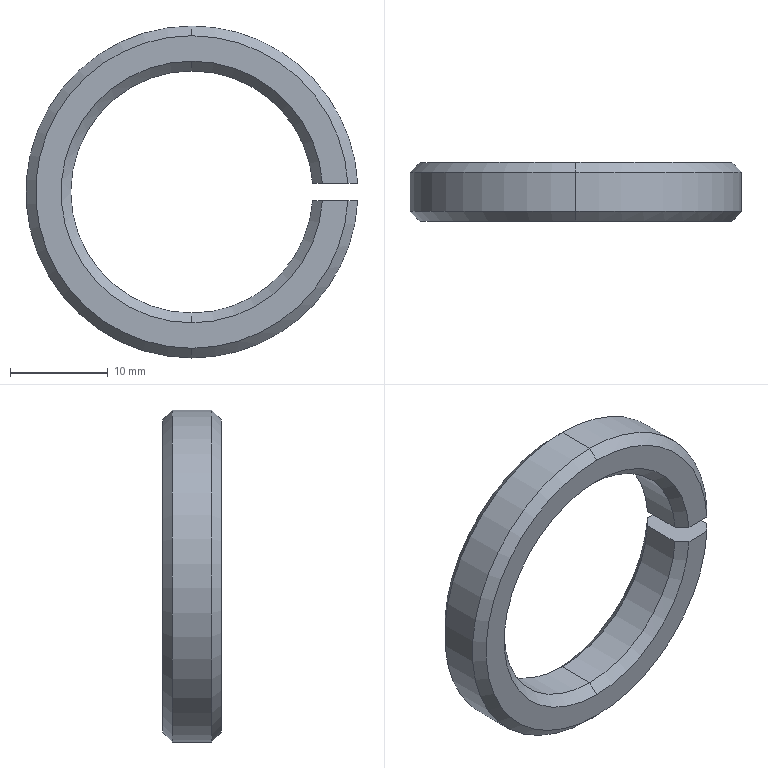Part | SolidWorks | mm | material Rubber | 1 solid | 22 faces | box 33.98 x 6 x 34 mm | volume 2318 mm3 | cone 12 | cylinder 6 | plane 4 | commonest cylinder face diameters 24.8 x3 34 x3
build123d program:
from build123d import *

# Parameters (mm, degrees)
SKETCH1_W          = 4.6
SKETCH1_H          = 6
CHAMFER1_SIZE      = 1
SKETCH2_W          = 15
SKETCH2_H          = 1.8
CUT_EXTRUDE1_DEPTH = 25.779


with BuildPart() as part:
    # Sketch1 → Revolve1 (revolve)
    with BuildSketch(Plane.XY, mode=Mode.PRIVATE) as revolve1_sk:
        with Locations((14.7, 0)):
            Rectangle(SKETCH1_W, SKETCH1_H)
    revolve(revolve1_sk.sketch.rotate(Axis((0, -27.466, 0), (0, 1, 0)), 90), axis=Axis((0, -27.466, 0), (0, 1, 0)))

    # Chamfer1
    chamfer1_edges = [part.edges().sort_by_distance(p)[0] for p in [
        (0, -3, 17),
        (0, -3, 12.4),
        (0, 3, 12.4),
        (0, 3, 17),
    ]]
    chamfer(chamfer1_edges, length=CHAMFER1_SIZE)

    # Sketch2 → Cut-Extrude1 (cut, through all)
    with BuildSketch(Plane(origin=(0, 3, 0), x_dir=(1, 0, 0), z_dir=(0, 1, 0))):
        with Locations((15.5, 0)):
            Rectangle(SKETCH2_W, SKETCH2_H)
    extrude(amount=-CUT_EXTRUDE1_DEPTH, mode=Mode.SUBTRACT)


solid = part.part
STEP:
#1=CARTESIAN_POINT('',(0.,3.,16.));
#2=VERTEX_POINT('',#1);
#3=CARTESIAN_POINT('',(15.975,3.,0.9));
#4=VERTEX_POINT('',#3);
#5=CARTESIAN_POINT('',(0.,3.,0.));
#6=DIRECTION('',(0.,1.,0.));
#7=DIRECTION('',(0.,0.,-1.));
#8=AXIS2_PLACEMENT_3D('',#5,#6,#7);
#9=CIRCLE('',#8,16.);
#10=EDGE_CURVE('',#2,#4,#9,.T.);
#11=ORIENTED_EDGE('',*,*,#10,.F.);
#12=CARTESIAN_POINT('',(0.,2.,17.));
#13=VERTEX_POINT('',#12);
#14=CARTESIAN_POINT('',(0.,2.,17.));
#15=DIRECTION('',(0.,-0.7071,0.7071));
#16=VECTOR('',#15,1000.);
#17=LINE('',#14,#16);
#18=EDGE_CURVE('',#2,#13,#17,.T.);
#19=ORIENTED_EDGE('',*,*,#18,.T.);
#20=CARTESIAN_POINT('',(16.976,2.,0.9));
#21=VERTEX_POINT('',#20);
#22=CARTESIAN_POINT('',(0.,2.,0.));
#23=DIRECTION('',(0.,-1.,0.));
#24=DIRECTION('',(0.,0.,-1.));
#25=AXIS2_PLACEMENT_3D('',#22,#23,#24);
#26=CIRCLE('',#25,17.);
#27=EDGE_CURVE('',#21,#13,#26,.T.);
#28=ORIENTED_EDGE('',*,*,#27,.F.);
#29=CARTESIAN_POINT('',(15.975,3.,0.9));
#30=CARTESIAN_POINT('',(16.309,2.667,0.9));
#31=CARTESIAN_POINT('',(16.642,2.333,0.9));
#32=CARTESIAN_POINT('',(16.976,2.,0.9));
#33=B_SPLINE_CURVE_WITH_KNOTS('',3,(#29,#30,#31,#32),.UNSPECIFIED.,.F.,.F.,(4,4),(0.01619,0.01761),.UNSPECIFIED.);
#34=EDGE_CURVE('',#4,#21,#33,.T.);
#35=ORIENTED_EDGE('',*,*,#34,.F.);
#36=EDGE_LOOP('',(#11,#19,#28,#35));
#37=FACE_OUTER_BOUND('',#36,.T.);
#38=CARTESIAN_POINT('',(0.,2.,0.));
#39=DIRECTION('',(0.,-1.,0.));
#40=DIRECTION('',(0.,0.,-1.));
#41=AXIS2_PLACEMENT_3D('',#38,#39,#40);
#42=CONICAL_SURFACE('',#41,17.,0.7854);
#43=ADVANCED_FACE('',(#37),#42,.T.);
#44=ORIENTED_EDGE('',*,*,#18,.F.);
#45=CARTESIAN_POINT('',(0.,3.,-16.));
#46=VERTEX_POINT('',#45);
#47=CARTESIAN_POINT('',(0.,3.,0.));
#48=DIRECTION('',(0.,1.,0.));
#49=DIRECTION('',(0.,0.,-1.));
#50=AXIS2_PLACEMENT_3D('',#47,#48,#49);
#51=CIRCLE('',#50,16.);
#52=EDGE_CURVE('',#46,#2,#51,.T.);
#53=ORIENTED_EDGE('',*,*,#52,.F.);
#54=CARTESIAN_POINT('',(0.,2.,-17.));
#55=VERTEX_POINT('',#54);
#56=CARTESIAN_POINT('',(0.,2.,-17.));
#57=DIRECTION('',(0.,-0.7071,-0.7071));
#58=VECTOR('',#57,1000.);
#59=LINE('',#56,#58);
#60=EDGE_CURVE('',#46,#55,#59,.T.);
#61=ORIENTED_EDGE('',*,*,#60,.T.);
#62=CARTESIAN_POINT('',(0.,2.,0.));
#63=DIRECTION('',(0.,-1.,0.));
#64=DIRECTION('',(0.,0.,-1.));
#65=AXIS2_PLACEMENT_3D('',#62,#63,#64);
#66=CIRCLE('',#65,17.);
#67=EDGE_CURVE('',#13,#55,#66,.T.);
#68=ORIENTED_EDGE('',*,*,#67,.F.);
#69=EDGE_LOOP('',(#44,#53,#61,#68));
#70=FACE_OUTER_BOUND('',#69,.T.);
#71=CARTESIAN_POINT('',(0.,2.,0.));
#72=DIRECTION('',(0.,-1.,0.));
#73=DIRECTION('',(0.,0.,-1.));
#74=AXIS2_PLACEMENT_3D('',#71,#72,#73);
#75=CONICAL_SURFACE('',#74,17.,0.7854);
#76=ADVANCED_FACE('',(#70),#75,.T.);
#77=CARTESIAN_POINT('',(0.,-3.,-16.));
#78=VERTEX_POINT('',#77);
#79=CARTESIAN_POINT('',(15.975,-3.,-0.9));
#80=VERTEX_POINT('',#79);
#81=CARTESIAN_POINT('',(0.,-3.,0.));
#82=DIRECTION('',(0.,-1.,0.));
#83=DIRECTION('',(0.,0.,-1.));
#84=AXIS2_PLACEMENT_3D('',#81,#82,#83);
#85=CIRCLE('',#84,16.);
#86=EDGE_CURVE('',#78,#80,#85,.T.);
#87=ORIENTED_EDGE('',*,*,#86,.F.);
#88=CARTESIAN_POINT('',(0.,-2.,-17.));
#89=VERTEX_POINT('',#88);
#90=CARTESIAN_POINT('',(0.,-3.,-16.));
#91=DIRECTION('',(0.,0.7071,-0.7071));
#92=VECTOR('',#91,1000.);
#93=LINE('',#90,#92);
#94=EDGE_CURVE('',#78,#89,#93,.T.);
#95=ORIENTED_EDGE('',*,*,#94,.T.);
#96=CARTESIAN_POINT('',(16.976,-2.,-0.9));
#97=VERTEX_POINT('',#96);
#98=CARTESIAN_POINT('',(0.,-2.,0.));
#99=DIRECTION('',(0.,1.,0.));
#100=DIRECTION('',(-0.,0.,-1.));
#101=AXIS2_PLACEMENT_3D('',#98,#99,#100);
#102=CIRCLE('',#101,17.);
#103=EDGE_CURVE('',#97,#89,#102,.T.);
#104=ORIENTED_EDGE('',*,*,#103,.F.);
#105=CARTESIAN_POINT('',(15.975,-3.,-0.9));
#106=CARTESIAN_POINT('',(16.309,-2.667,-0.9));
#107=CARTESIAN_POINT('',(16.642,-2.333,-0.9));
#108=CARTESIAN_POINT('',(16.976,-2.,-0.9));
#109=B_SPLINE_CURVE_WITH_KNOTS('',3,(#105,#106,#107,#108),.UNSPECIFIED.,.F.,.F.,(4,4),(0.01619,0.01761),.UNSPECIFIED.);
#110=EDGE_CURVE('',#80,#97,#109,.T.);
#111=ORIENTED_EDGE('',*,*,#110,.F.);
#112=EDGE_LOOP('',(#87,#95,#104,#111));
#113=FACE_OUTER_BOUND('',#112,.T.);
#114=CARTESIAN_POINT('',(0.,-3.,0.));
#115=DIRECTION('',(0.,1.,0.));
#116=DIRECTION('',(0.,0.,1.));
#117=AXIS2_PLACEMENT_3D('',#114,#115,#116);
#118=CONICAL_SURFACE('',#117,16.,0.7854);
#119=ADVANCED_FACE('',(#113),#118,.T.);
#120=ORIENTED_EDGE('',*,*,#94,.F.);
#121=CARTESIAN_POINT('',(0.,-3.,16.));
#122=VERTEX_POINT('',#121);
#123=CARTESIAN_POINT('',(0.,-3.,0.));
#124=DIRECTION('',(0.,-1.,0.));
#125=DIRECTION('',(0.,0.,-1.));
#126=AXIS2_PLACEMENT_3D('',#123,#124,#125);
#127=CIRCLE('',#126,16.);
#128=EDGE_CURVE('',#122,#78,#127,.T.);
#129=ORIENTED_EDGE('',*,*,#128,.F.);
#130=CARTESIAN_POINT('',(0.,-2.,17.));
#131=VERTEX_POINT('',#130);
#132=CARTESIAN_POINT('',(0.,-3.,16.));
#133=DIRECTION('',(0.,0.7071,0.7071));
#134=VECTOR('',#133,1000.);
#135=LINE('',#132,#134);
#136=EDGE_CURVE('',#122,#131,#135,.T.);
#137=ORIENTED_EDGE('',*,*,#136,.T.);
#138=CARTESIAN_POINT('',(0.,-2.,0.));
#139=DIRECTION('',(0.,1.,0.));
#140=DIRECTION('',(0.,0.,-1.));
#141=AXIS2_PLACEMENT_3D('',#138,#139,#140);
#142=CIRCLE('',#141,17.);
#143=EDGE_CURVE('',#89,#131,#142,.T.);
#144=ORIENTED_EDGE('',*,*,#143,.F.);
#145=EDGE_LOOP('',(#120,#129,#137,#144));
#146=FACE_OUTER_BOUND('',#145,.T.);
#147=CARTESIAN_POINT('',(0.,-3.,0.));
#148=DIRECTION('',(0.,1.,0.));
#149=DIRECTION('',(0.,0.,1.));
#150=AXIS2_PLACEMENT_3D('',#147,#148,#149);
#151=CONICAL_SURFACE('',#150,16.,0.7854);
#152=ADVANCED_FACE('',(#146),#151,.T.);
#153=CARTESIAN_POINT('',(0.,2.,-12.4));
#154=VERTEX_POINT('',#153);
#155=CARTESIAN_POINT('',(0.,2.,12.4));
#156=VERTEX_POINT('',#155);
#157=CARTESIAN_POINT('',(0.,2.,0.));
#158=DIRECTION('',(0.,1.,0.));
#159=DIRECTION('',(0.,0.,-1.));
#160=AXIS2_PLACEMENT_3D('',#157,#158,#159);
#161=CIRCLE('',#160,12.4);
#162=EDGE_CURVE('',#154,#156,#161,.T.);
#163=ORIENTED_EDGE('',*,*,#162,.F.);
#164=CARTESIAN_POINT('',(0.,3.,-13.4));
#165=VERTEX_POINT('',#164);
#166=CARTESIAN_POINT('',(0.,3.,-13.4));
#167=DIRECTION('',(0.,0.7071,-0.7071));
#168=VECTOR('',#167,1000.);
#169=LINE('',#166,#168);
#170=EDGE_CURVE('',#154,#165,#169,.T.);
#171=ORIENTED_EDGE('',*,*,#170,.T.);
#172=CARTESIAN_POINT('',(0.,3.,13.4));
#173=VERTEX_POINT('',#172);
#174=CARTESIAN_POINT('',(0.,3.,0.));
#175=DIRECTION('',(0.,-1.,0.));
#176=DIRECTION('',(0.,0.,-1.));
#177=AXIS2_PLACEMENT_3D('',#174,#175,#176);
#178=CIRCLE('',#177,13.4);
#179=EDGE_CURVE('',#173,#165,#178,.T.);
#180=ORIENTED_EDGE('',*,*,#179,.F.);
#181=CARTESIAN_POINT('',(0.,3.,13.4));
#182=DIRECTION('',(0.,0.7071,0.7071));
#183=VECTOR('',#182,1000.);
#184=LINE('',#181,#183);
#185=EDGE_CURVE('',#156,#173,#184,.T.);
#186=ORIENTED_EDGE('',*,*,#185,.F.);
#187=EDGE_LOOP('',(#163,#171,#180,#186));
#188=FACE_OUTER_BOUND('',#187,.T.);
#189=CARTESIAN_POINT('',(0.,3.,0.));
#190=DIRECTION('',(0.,1.,0.));
#191=DIRECTION('',(0.,0.,1.));
#192=AXIS2_PLACEMENT_3D('',#189,#190,#191);
#193=CONICAL_SURFACE('',#192,13.4,0.7854);
#194=ADVANCED_FACE('',(#188),#193,.F.);
#195=CARTESIAN_POINT('',(12.367,2.,0.9));
#196=VERTEX_POINT('',#195);
#197=CARTESIAN_POINT('',(0.,2.,0.));
#198=DIRECTION('',(0.,1.,0.));
#199=DIRECTION('',(0.,0.,-1.));
#200=AXIS2_PLACEMENT_3D('',#197,#198,#199);
#201=CIRCLE('',#200,12.4);
#202=EDGE_CURVE('',#156,#196,#201,.T.);
#203=ORIENTED_EDGE('',*,*,#202,.F.);
#204=ORIENTED_EDGE('',*,*,#185,.T.);
#205=CARTESIAN_POINT('',(13.37,3.,0.9));
#206=VERTEX_POINT('',#205);
#207=CARTESIAN_POINT('',(0.,3.,0.));
#208=DIRECTION('',(0.,-1.,0.));
#209=DIRECTION('',(0.,0.,-1.));
#210=AXIS2_PLACEMENT_3D('',#207,#208,#209);
#211=CIRCLE('',#210,13.4);
#212=EDGE_CURVE('',#206,#173,#211,.T.);
#213=ORIENTED_EDGE('',*,*,#212,.F.);
#214=CARTESIAN_POINT('',(12.367,2.,0.9));
#215=CARTESIAN_POINT('',(12.701,2.333,0.9));
#216=CARTESIAN_POINT('',(13.036,2.667,0.9));
#217=CARTESIAN_POINT('',(13.37,3.,0.9));
#218=B_SPLINE_CURVE_WITH_KNOTS('',3,(#214,#215,#216,#217),.UNSPECIFIED.,.F.,.F.,(4,4),(0.009566,0.01098),.UNSPECIFIED.);
#219=EDGE_CURVE('',#196,#206,#218,.T.);
#220=ORIENTED_EDGE('',*,*,#219,.F.);
#221=EDGE_LOOP('',(#203,#204,#213,#220));
#222=FACE_OUTER_BOUND('',#221,.T.);
#223=CARTESIAN_POINT('',(0.,3.,0.));
#224=DIRECTION('',(0.,1.,0.));
#225=DIRECTION('',(0.,0.,1.));
#226=AXIS2_PLACEMENT_3D('',#223,#224,#225);
#227=CONICAL_SURFACE('',#226,13.4,0.7854);
#228=ADVANCED_FACE('',(#222),#227,.F.);
#229=CARTESIAN_POINT('',(0.,-2.,12.4));
#230=VERTEX_POINT('',#229);
#231=CARTESIAN_POINT('',(0.,-2.,-12.4));
#232=VERTEX_POINT('',#231);
#233=CARTESIAN_POINT('',(0.,-2.,0.));
#234=DIRECTION('',(0.,-1.,0.));
#235=DIRECTION('',(0.,0.,-1.));
#236=AXIS2_PLACEMENT_3D('',#233,#234,#235);
#237=CIRCLE('',#236,12.4);
#238=EDGE_CURVE('',#230,#232,#237,.T.);
#239=ORIENTED_EDGE('',*,*,#238,.F.);
#240=CARTESIAN_POINT('',(0.,-3.,13.4));
#241=VERTEX_POINT('',#240);
#242=CARTESIAN_POINT('',(0.,-2.,12.4));
#243=DIRECTION('',(0.,-0.7071,0.7071));
#244=VECTOR('',#243,1000.);
#245=LINE('',#242,#244);
#246=EDGE_CURVE('',#230,#241,#245,.T.);
#247=ORIENTED_EDGE('',*,*,#246,.T.);
#248=CARTESIAN_POINT('',(0.,-3.,-13.4));
#249=VERTEX_POINT('',#248);
#250=CARTESIAN_POINT('',(0.,-3.,0.));
#251=DIRECTION('',(0.,1.,0.));
#252=DIRECTION('',(0.,0.,-1.));
#253=AXIS2_PLACEMENT_3D('',#250,#251,#252);
#254=CIRCLE('',#253,13.4);
#255=EDGE_CURVE('',#249,#241,#254,.T.);
#256=ORIENTED_EDGE('',*,*,#255,.F.);
#257=CARTESIAN_POINT('',(0.,-2.,-12.4));
#258=DIRECTION('',(0.,-0.7071,-0.7071));
#259=VECTOR('',#258,1000.);
#260=LINE('',#257,#259);
#261=EDGE_CURVE('',#232,#249,#260,.T.);
#262=ORIENTED_EDGE('',*,*,#261,.F.);
#263=EDGE_LOOP('',(#239,#247,#256,#262));
#264=FACE_OUTER_BOUND('',#263,.T.);
#265=CARTESIAN_POINT('',(0.,-2.,0.));
#266=DIRECTION('',(0.,-1.,0.));
#267=DIRECTION('',(0.,0.,-1.));
#268=AXIS2_PLACEMENT_3D('',#265,#266,#267);
#269=CONICAL_SURFACE('',#268,12.4,0.7854);
#270=ADVANCED_FACE('',(#264),#269,.F.);
#271=CARTESIAN_POINT('',(12.367,-2.,-0.9));
#272=VERTEX_POINT('',#271);
#273=CARTESIAN_POINT('',(0.,-2.,0.));
#274=DIRECTION('',(0.,-1.,0.));
#275=DIRECTION('',(0.,0.,-1.));
#276=AXIS2_PLACEMENT_3D('',#273,#274,#275);
#277=CIRCLE('',#276,12.4);
#278=EDGE_CURVE('',#232,#272,#277,.T.);
#279=ORIENTED_EDGE('',*,*,#278,.F.);
#280=ORIENTED_EDGE('',*,*,#261,.T.);
#281=CARTESIAN_POINT('',(13.37,-3.,-0.9));
#282=VERTEX_POINT('',#281);
#283=CARTESIAN_POINT('',(0.,-3.,0.));
#284=DIRECTION('',(0.,1.,0.));
#285=DIRECTION('',(-0.,0.,-1.));
#286=AXIS2_PLACEMENT_3D('',#283,#284,#285);
#287=CIRCLE('',#286,13.4);
#288=EDGE_CURVE('',#282,#249,#287,.T.);
#289=ORIENTED_EDGE('',*,*,#288,.F.);
#290=CARTESIAN_POINT('',(12.367,-2.,-0.9));
#291=CARTESIAN_POINT('',(12.701,-2.333,-0.9));
#292=CARTESIAN_POINT('',(13.036,-2.667,-0.9));
#293=CARTESIAN_POINT('',(13.37,-3.,-0.9));
#294=B_SPLINE_CURVE_WITH_KNOTS('',3,(#290,#291,#292,#293),.UNSPECIFIED.,.F.,.F.,(4,4),(0.009566,0.01098),.UNSPECIFIED.);
#295=EDGE_CURVE('',#272,#282,#294,.T.);
#296=ORIENTED_EDGE('',*,*,#295,.F.);
#297=EDGE_LOOP('',(#279,#280,#289,#296));
#298=FACE_OUTER_BOUND('',#297,.T.);
#299=CARTESIAN_POINT('',(0.,-2.,0.));
#300=DIRECTION('',(0.,-1.,0.));
#301=DIRECTION('',(0.,0.,-1.));
#302=AXIS2_PLACEMENT_3D('',#299,#300,#301);
#303=CONICAL_SURFACE('',#302,12.4,0.7854);
#304=ADVANCED_FACE('',(#298),#303,.F.);
#305=ORIENTED_EDGE('',*,*,#162,.T.);
#306=CARTESIAN_POINT('',(0.,-27.466,12.4));
#307=DIRECTION('',(0.,-1.,0.));
#308=VECTOR('',#307,1000.);
#309=LINE('',#306,#308);
#310=EDGE_CURVE('',#156,#230,#309,.T.);
#311=ORIENTED_EDGE('',*,*,#310,.T.);
#312=ORIENTED_EDGE('',*,*,#238,.T.);
#313=CARTESIAN_POINT('',(0.,-27.466,-12.4));
#314=DIRECTION('',(0.,-1.,0.));
#315=VECTOR('',#314,1000.);
#316=LINE('',#313,#315);
#317=EDGE_CURVE('',#154,#232,#316,.T.);
#318=ORIENTED_EDGE('',*,*,#317,.F.);
#319=EDGE_LOOP('',(#305,#311,#312,#318));
#320=FACE_OUTER_BOUND('',#319,.T.);
#321=CARTESIAN_POINT('',(0.,-27.466,0.));
#322=DIRECTION('',(0.,-1.,0.));
#323=DIRECTION('',(0.,0.,-1.));
#324=AXIS2_PLACEMENT_3D('',#321,#322,#323);
#325=CYLINDRICAL_SURFACE('',#324,12.4);
#326=ADVANCED_FACE('',(#320),#325,.F.);
#327=CARTESIAN_POINT('',(12.367,2.,-0.9));
#328=VERTEX_POINT('',#327);
#329=CARTESIAN_POINT('',(0.,2.,0.));
#330=DIRECTION('',(0.,1.,0.));
#331=DIRECTION('',(-0.,0.,-1.));
#332=AXIS2_PLACEMENT_3D('',#329,#330,#331);
#333=CIRCLE('',#332,12.4);
#334=EDGE_CURVE('',#328,#154,#333,.T.);
#335=ORIENTED_EDGE('',*,*,#334,.T.);
#336=ORIENTED_EDGE('',*,*,#317,.T.);
#337=ORIENTED_EDGE('',*,*,#278,.T.);
#338=CARTESIAN_POINT('',(12.367,-27.466,-0.9));
#339=DIRECTION('',(0.,-1.,0.));
#340=VECTOR('',#339,1000.);
#341=LINE('',#338,#340);
#342=EDGE_CURVE('',#328,#272,#341,.T.);
#343=ORIENTED_EDGE('',*,*,#342,.F.);
#344=EDGE_LOOP('',(#335,#336,#337,#343));
#345=FACE_OUTER_BOUND('',#344,.T.);
#346=CARTESIAN_POINT('',(0.,-27.466,0.));
#347=DIRECTION('',(0.,-1.,0.));
#348=DIRECTION('',(0.,0.,-1.));
#349=AXIS2_PLACEMENT_3D('',#346,#347,#348);
#350=CYLINDRICAL_SURFACE('',#349,12.4);
#351=ADVANCED_FACE('',(#345),#350,.F.);
#352=ORIENTED_EDGE('',*,*,#27,.T.);
#353=CARTESIAN_POINT('',(0.,-27.466,17.));
#354=DIRECTION('',(0.,-1.,0.));
#355=VECTOR('',#354,1000.);
#356=LINE('',#353,#355);
#357=EDGE_CURVE('',#13,#131,#356,.T.);
#358=ORIENTED_EDGE('',*,*,#357,.T.);
#359=CARTESIAN_POINT('',(16.976,-2.,0.9));
#360=VERTEX_POINT('',#359);
#361=CARTESIAN_POINT('',(0.,-2.,0.));
#362=DIRECTION('',(0.,1.,0.));
#363=DIRECTION('',(0.,0.,-1.));
#364=AXIS2_PLACEMENT_3D('',#361,#362,#363);
#365=CIRCLE('',#364,17.);
#366=EDGE_CURVE('',#131,#360,#365,.T.);
#367=ORIENTED_EDGE('',*,*,#366,.T.);
#368=CARTESIAN_POINT('',(16.976,-27.466,0.9));
#369=DIRECTION('',(0.,1.,0.));
#370=VECTOR('',#369,1000.);
#371=LINE('',#368,#370);
#372=EDGE_CURVE('',#360,#21,#371,.T.);
#373=ORIENTED_EDGE('',*,*,#372,.T.);
#374=EDGE_LOOP('',(#352,#358,#367,#373));
#375=FACE_OUTER_BOUND('',#374,.T.);
#376=CARTESIAN_POINT('',(0.,-27.466,0.));
#377=DIRECTION('',(0.,-1.,0.));
#378=DIRECTION('',(0.,0.,-1.));
#379=AXIS2_PLACEMENT_3D('',#376,#377,#378);
#380=CYLINDRICAL_SURFACE('',#379,17.);
#381=ADVANCED_FACE('',(#375),#380,.T.);
#382=ORIENTED_EDGE('',*,*,#357,.F.);
#383=ORIENTED_EDGE('',*,*,#67,.T.);
#384=CARTESIAN_POINT('',(0.,-27.466,-17.));
#385=DIRECTION('',(0.,-1.,0.));
#386=VECTOR('',#385,1000.);
#387=LINE('',#384,#386);
#388=EDGE_CURVE('',#55,#89,#387,.T.);
#389=ORIENTED_EDGE('',*,*,#388,.T.);
#390=ORIENTED_EDGE('',*,*,#143,.T.);
#391=EDGE_LOOP('',(#382,#383,#389,#390));
#392=FACE_OUTER_BOUND('',#391,.T.);
#393=CARTESIAN_POINT('',(0.,-27.466,0.));
#394=DIRECTION('',(0.,-1.,0.));
#395=DIRECTION('',(0.,0.,-1.));
#396=AXIS2_PLACEMENT_3D('',#393,#394,#395);
#397=CYLINDRICAL_SURFACE('',#396,17.);
#398=ADVANCED_FACE('',(#392),#397,.T.);
#399=ORIENTED_EDGE('',*,*,#388,.F.);
#400=CARTESIAN_POINT('',(16.976,2.,-0.9));
#401=VERTEX_POINT('',#400);
#402=CARTESIAN_POINT('',(0.,2.,0.));
#403=DIRECTION('',(0.,-1.,0.));
#404=DIRECTION('',(0.,0.,-1.));
#405=AXIS2_PLACEMENT_3D('',#402,#403,#404);
#406=CIRCLE('',#405,17.);
#407=EDGE_CURVE('',#55,#401,#406,.T.);
#408=ORIENTED_EDGE('',*,*,#407,.T.);
#409=CARTESIAN_POINT('',(16.976,-27.466,-0.9));
#410=DIRECTION('',(0.,-1.,0.));
#411=VECTOR('',#410,1000.);
#412=LINE('',#409,#411);
#413=EDGE_CURVE('',#401,#97,#412,.T.);
#414=ORIENTED_EDGE('',*,*,#413,.T.);
#415=ORIENTED_EDGE('',*,*,#103,.T.);
#416=EDGE_LOOP('',(#399,#408,#414,#415));
#417=FACE_OUTER_BOUND('',#416,.T.);
#418=CARTESIAN_POINT('',(0.,-27.466,0.));
#419=DIRECTION('',(0.,-1.,0.));
#420=DIRECTION('',(0.,0.,-1.));
#421=AXIS2_PLACEMENT_3D('',#418,#419,#420);
#422=CYLINDRICAL_SURFACE('',#421,17.);
#423=ADVANCED_FACE('',(#417),#422,.T.);
#424=ORIENTED_EDGE('',*,*,#212,.T.);
#425=ORIENTED_EDGE('',*,*,#179,.T.);
#426=CARTESIAN_POINT('',(13.37,3.,-0.9));
#427=VERTEX_POINT('',#426);
#428=CARTESIAN_POINT('',(0.,3.,0.));
#429=DIRECTION('',(0.,-1.,0.));
#430=DIRECTION('',(0.,0.,-1.));
#431=AXIS2_PLACEMENT_3D('',#428,#429,#430);
#432=CIRCLE('',#431,13.4);
#433=EDGE_CURVE('',#165,#427,#432,.T.);
#434=ORIENTED_EDGE('',*,*,#433,.T.);
#435=CARTESIAN_POINT('',(15.975,3.,-0.9));
#436=VERTEX_POINT('',#435);
#437=CARTESIAN_POINT('',(8.,3.,-0.9));
#438=DIRECTION('',(-1.,0.,0.));
#439=VECTOR('',#438,1000.);
#440=LINE('',#437,#439);
#441=EDGE_CURVE('',#436,#427,#440,.T.);
#442=ORIENTED_EDGE('',*,*,#441,.F.);
#443=CARTESIAN_POINT('',(0.,3.,0.));
#444=DIRECTION('',(0.,1.,0.));
#445=DIRECTION('',(-0.,0.,-1.));
#446=AXIS2_PLACEMENT_3D('',#443,#444,#445);
#447=CIRCLE('',#446,16.);
#448=EDGE_CURVE('',#436,#46,#447,.T.);
#449=ORIENTED_EDGE('',*,*,#448,.T.);
#450=ORIENTED_EDGE('',*,*,#52,.T.);
#451=ORIENTED_EDGE('',*,*,#10,.T.);
#452=CARTESIAN_POINT('',(8.,3.,0.9));
#453=DIRECTION('',(1.,0.,0.));
#454=VECTOR('',#453,1000.);
#455=LINE('',#452,#454);
#456=EDGE_CURVE('',#206,#4,#455,.T.);
#457=ORIENTED_EDGE('',*,*,#456,.F.);
#458=EDGE_LOOP('',(#424,#425,#434,#442,#449,#450,#451,#457));
#459=FACE_OUTER_BOUND('',#458,.T.);
#460=CARTESIAN_POINT('',(0.,3.,0.));
#461=DIRECTION('',(0.,-1.,0.));
#462=DIRECTION('',(0.,0.,-1.));
#463=AXIS2_PLACEMENT_3D('',#460,#461,#462);
#464=PLANE('',#463);
#465=ADVANCED_FACE('',(#459),#464,.F.);
#466=ORIENTED_EDGE('',*,*,#310,.F.);
#467=ORIENTED_EDGE('',*,*,#202,.T.);
#468=CARTESIAN_POINT('',(12.367,-2.,0.9));
#469=VERTEX_POINT('',#468);
#470=CARTESIAN_POINT('',(12.367,-27.466,0.9));
#471=DIRECTION('',(0.,1.,0.));
#472=VECTOR('',#471,1000.);
#473=LINE('',#470,#472);
#474=EDGE_CURVE('',#469,#196,#473,.T.);
#475=ORIENTED_EDGE('',*,*,#474,.F.);
#476=CARTESIAN_POINT('',(0.,-2.,0.));
#477=DIRECTION('',(0.,-1.,0.));
#478=DIRECTION('',(0.,0.,-1.));
#479=AXIS2_PLACEMENT_3D('',#476,#477,#478);
#480=CIRCLE('',#479,12.4);
#481=EDGE_CURVE('',#469,#230,#480,.T.);
#482=ORIENTED_EDGE('',*,*,#481,.T.);
#483=EDGE_LOOP('',(#466,#467,#475,#482));
#484=FACE_OUTER_BOUND('',#483,.T.);
#485=CARTESIAN_POINT('',(0.,-27.466,0.));
#486=DIRECTION('',(0.,-1.,0.));
#487=DIRECTION('',(0.,0.,-1.));
#488=AXIS2_PLACEMENT_3D('',#485,#486,#487);
#489=CYLINDRICAL_SURFACE('',#488,12.4);
#490=ADVANCED_FACE('',(#484),#489,.F.);
#491=CARTESIAN_POINT('',(8.,-3.,-0.9));
#492=DIRECTION('',(-1.,0.,0.));
#493=VECTOR('',#492,1000.);
#494=LINE('',#491,#493);
#495=EDGE_CURVE('',#80,#282,#494,.T.);
#496=ORIENTED_EDGE('',*,*,#495,.T.);
#497=ORIENTED_EDGE('',*,*,#288,.T.);
#498=ORIENTED_EDGE('',*,*,#255,.T.);
#499=CARTESIAN_POINT('',(13.37,-3.,0.9));
#500=VERTEX_POINT('',#499);
#501=CARTESIAN_POINT('',(0.,-3.,0.));
#502=DIRECTION('',(0.,1.,0.));
#503=DIRECTION('',(0.,0.,-1.));
#504=AXIS2_PLACEMENT_3D('',#501,#502,#503);
#505=CIRCLE('',#504,13.4);
#506=EDGE_CURVE('',#241,#500,#505,.T.);
#507=ORIENTED_EDGE('',*,*,#506,.T.);
#508=CARTESIAN_POINT('',(15.975,-3.,0.9));
#509=VERTEX_POINT('',#508);
#510=CARTESIAN_POINT('',(8.,-3.,0.9));
#511=DIRECTION('',(1.,0.,0.));
#512=VECTOR('',#511,1000.);
#513=LINE('',#510,#512);
#514=EDGE_CURVE('',#500,#509,#513,.T.);
#515=ORIENTED_EDGE('',*,*,#514,.T.);
#516=CARTESIAN_POINT('',(0.,-3.,0.));
#517=DIRECTION('',(0.,-1.,0.));
#518=DIRECTION('',(0.,0.,-1.));
#519=AXIS2_PLACEMENT_3D('',#516,#517,#518);
#520=CIRCLE('',#519,16.);
#521=EDGE_CURVE('',#509,#122,#520,.T.);
#522=ORIENTED_EDGE('',*,*,#521,.T.);
#523=ORIENTED_EDGE('',*,*,#128,.T.);
#524=ORIENTED_EDGE('',*,*,#86,.T.);
#525=EDGE_LOOP('',(#496,#497,#498,#507,#515,#522,#523,#524));
#526=FACE_OUTER_BOUND('',#525,.T.);
#527=CARTESIAN_POINT('',(0.,-3.,0.));
#528=DIRECTION('',(0.,-1.,0.));
#529=DIRECTION('',(0.,0.,-1.));
#530=AXIS2_PLACEMENT_3D('',#527,#528,#529);
#531=PLANE('',#530);
#532=ADVANCED_FACE('',(#526),#531,.T.);
#533=ORIENTED_EDGE('',*,*,#246,.F.);
#534=ORIENTED_EDGE('',*,*,#481,.F.);
#535=CARTESIAN_POINT('',(13.37,-3.,0.9));
#536=CARTESIAN_POINT('',(13.036,-2.667,0.9));
#537=CARTESIAN_POINT('',(12.701,-2.333,0.9));
#538=CARTESIAN_POINT('',(12.367,-2.,0.9));
#539=B_SPLINE_CURVE_WITH_KNOTS('',3,(#535,#536,#537,#538),.UNSPECIFIED.,.F.,.F.,(4,4),(0.009363,0.01078),.UNSPECIFIED.);
#540=EDGE_CURVE('',#500,#469,#539,.T.);
#541=ORIENTED_EDGE('',*,*,#540,.F.);
#542=ORIENTED_EDGE('',*,*,#506,.F.);
#543=EDGE_LOOP('',(#533,#534,#541,#542));
#544=FACE_OUTER_BOUND('',#543,.T.);
#545=CARTESIAN_POINT('',(0.,-2.,0.));
#546=DIRECTION('',(0.,-1.,0.));
#547=DIRECTION('',(0.,0.,-1.));
#548=AXIS2_PLACEMENT_3D('',#545,#546,#547);
#549=CONICAL_SURFACE('',#548,12.4,0.7854);
#550=ADVANCED_FACE('',(#544),#549,.F.);
#551=ORIENTED_EDGE('',*,*,#170,.F.);
#552=ORIENTED_EDGE('',*,*,#334,.F.);
#553=CARTESIAN_POINT('',(13.37,3.,-0.9));
#554=CARTESIAN_POINT('',(13.036,2.667,-0.9));
#555=CARTESIAN_POINT('',(12.701,2.333,-0.9));
#556=CARTESIAN_POINT('',(12.367,2.,-0.9));
#557=B_SPLINE_CURVE_WITH_KNOTS('',3,(#553,#554,#555,#556),.UNSPECIFIED.,.F.,.F.,(4,4),(0.009363,0.01078),.UNSPECIFIED.);
#558=EDGE_CURVE('',#427,#328,#557,.T.);
#559=ORIENTED_EDGE('',*,*,#558,.F.);
#560=ORIENTED_EDGE('',*,*,#433,.F.);
#561=EDGE_LOOP('',(#551,#552,#559,#560));
#562=FACE_OUTER_BOUND('',#561,.T.);
#563=CARTESIAN_POINT('',(0.,3.,0.));
#564=DIRECTION('',(0.,1.,0.));
#565=DIRECTION('',(0.,0.,1.));
#566=AXIS2_PLACEMENT_3D('',#563,#564,#565);
#567=CONICAL_SURFACE('',#566,13.4,0.7854);
#568=ADVANCED_FACE('',(#562),#567,.F.);
#569=ORIENTED_EDGE('',*,*,#136,.F.);
#570=ORIENTED_EDGE('',*,*,#521,.F.);
#571=CARTESIAN_POINT('',(16.976,-2.,0.9));
#572=CARTESIAN_POINT('',(16.642,-2.333,0.9));
#573=CARTESIAN_POINT('',(16.309,-2.667,0.9));
#574=CARTESIAN_POINT('',(15.975,-3.,0.9));
#575=B_SPLINE_CURVE_WITH_KNOTS('',3,(#571,#572,#573,#574),.UNSPECIFIED.,.F.,.F.,(4,4),(0.01534,0.01676),.UNSPECIFIED.);
#576=EDGE_CURVE('',#360,#509,#575,.T.);
#577=ORIENTED_EDGE('',*,*,#576,.F.);
#578=ORIENTED_EDGE('',*,*,#366,.F.);
#579=EDGE_LOOP('',(#569,#570,#577,#578));
#580=FACE_OUTER_BOUND('',#579,.T.);
#581=CARTESIAN_POINT('',(0.,-3.,0.));
#582=DIRECTION('',(0.,1.,0.));
#583=DIRECTION('',(0.,0.,1.));
#584=AXIS2_PLACEMENT_3D('',#581,#582,#583);
#585=CONICAL_SURFACE('',#584,16.,0.7854);
#586=ADVANCED_FACE('',(#580),#585,.T.);
#587=ORIENTED_EDGE('',*,*,#60,.F.);
#588=ORIENTED_EDGE('',*,*,#448,.F.);
#589=CARTESIAN_POINT('',(16.976,2.,-0.9));
#590=CARTESIAN_POINT('',(16.642,2.333,-0.9));
#591=CARTESIAN_POINT('',(16.309,2.667,-0.9));
#592=CARTESIAN_POINT('',(15.975,3.,-0.9));
#593=B_SPLINE_CURVE_WITH_KNOTS('',3,(#589,#590,#591,#592),.UNSPECIFIED.,.F.,.F.,(4,4),(0.01534,0.01676),.UNSPECIFIED.);
#594=EDGE_CURVE('',#401,#436,#593,.T.);
#595=ORIENTED_EDGE('',*,*,#594,.F.);
#596=ORIENTED_EDGE('',*,*,#407,.F.);
#597=EDGE_LOOP('',(#587,#588,#595,#596));
#598=FACE_OUTER_BOUND('',#597,.T.);
#599=CARTESIAN_POINT('',(0.,2.,0.));
#600=DIRECTION('',(0.,-1.,0.));
#601=DIRECTION('',(0.,0.,-1.));
#602=AXIS2_PLACEMENT_3D('',#599,#600,#601);
#603=CONICAL_SURFACE('',#602,17.,0.7854);
#604=ADVANCED_FACE('',(#598),#603,.T.);
#605=ORIENTED_EDGE('',*,*,#540,.T.);
#606=ORIENTED_EDGE('',*,*,#474,.T.);
#607=ORIENTED_EDGE('',*,*,#219,.T.);
#608=ORIENTED_EDGE('',*,*,#456,.T.);
#609=ORIENTED_EDGE('',*,*,#34,.T.);
#610=ORIENTED_EDGE('',*,*,#372,.F.);
#611=ORIENTED_EDGE('',*,*,#576,.T.);
#612=ORIENTED_EDGE('',*,*,#514,.F.);
#613=EDGE_LOOP('',(#605,#606,#607,#608,#609,#610,#611,#612));
#614=FACE_OUTER_BOUND('',#613,.T.);
#615=CARTESIAN_POINT('',(8.,-3.,0.9));
#616=DIRECTION('',(0.,0.,1.));
#617=DIRECTION('',(1.,0.,0.));
#618=AXIS2_PLACEMENT_3D('',#615,#616,#617);
#619=PLANE('',#618);
#620=ADVANCED_FACE('',(#614),#619,.F.);
#621=ORIENTED_EDGE('',*,*,#295,.T.);
#622=ORIENTED_EDGE('',*,*,#495,.F.);
#623=ORIENTED_EDGE('',*,*,#110,.T.);
#624=ORIENTED_EDGE('',*,*,#413,.F.);
#625=ORIENTED_EDGE('',*,*,#594,.T.);
#626=ORIENTED_EDGE('',*,*,#441,.T.);
#627=ORIENTED_EDGE('',*,*,#558,.T.);
#628=ORIENTED_EDGE('',*,*,#342,.T.);
#629=EDGE_LOOP('',(#621,#622,#623,#624,#625,#626,#627,#628));
#630=FACE_OUTER_BOUND('',#629,.T.);
#631=CARTESIAN_POINT('',(8.,-3.,-0.9));
#632=DIRECTION('',(0.,0.,-1.));
#633=DIRECTION('',(-1.,0.,0.));
#634=AXIS2_PLACEMENT_3D('',#631,#632,#633);
#635=PLANE('',#634);
#636=ADVANCED_FACE('',(#630),#635,.F.);
#637=CLOSED_SHELL('',(#43,#76,#119,#152,#194,#228,#270,#304,#326,#351,#381,#398,#423,#465,#490,#532,#550,#568,#586,#604,#620,#636));
#638=MANIFOLD_SOLID_BREP('',#637);
#639=CARTESIAN_POINT('',(0.,0.,0.));
#640=DIRECTION('',(0.,0.,1.));
#641=DIRECTION('',(1.,0.,0.));
#642=AXIS2_PLACEMENT_3D('',#639,#640,#641);
#643=(LENGTH_UNIT()NAMED_UNIT(*)SI_UNIT(.MILLI.,.METRE.));
#644=UNCERTAINTY_MEASURE_WITH_UNIT(LENGTH_MEASURE(0.00001),#643,'','');
#645=(NAMED_UNIT(*)PLANE_ANGLE_UNIT()SI_UNIT($,.RADIAN.));
#646=(NAMED_UNIT(*)SI_UNIT($,.STERADIAN.)SOLID_ANGLE_UNIT());
#647=(GEOMETRIC_REPRESENTATION_CONTEXT(3)GLOBAL_UNCERTAINTY_ASSIGNED_CONTEXT((#644))GLOBAL_UNIT_ASSIGNED_CONTEXT((#643,#645,#646))REPRESENTATION_CONTEXT('',''));
#648=ADVANCED_BREP_SHAPE_REPRESENTATION('',(#638,#642),#647);